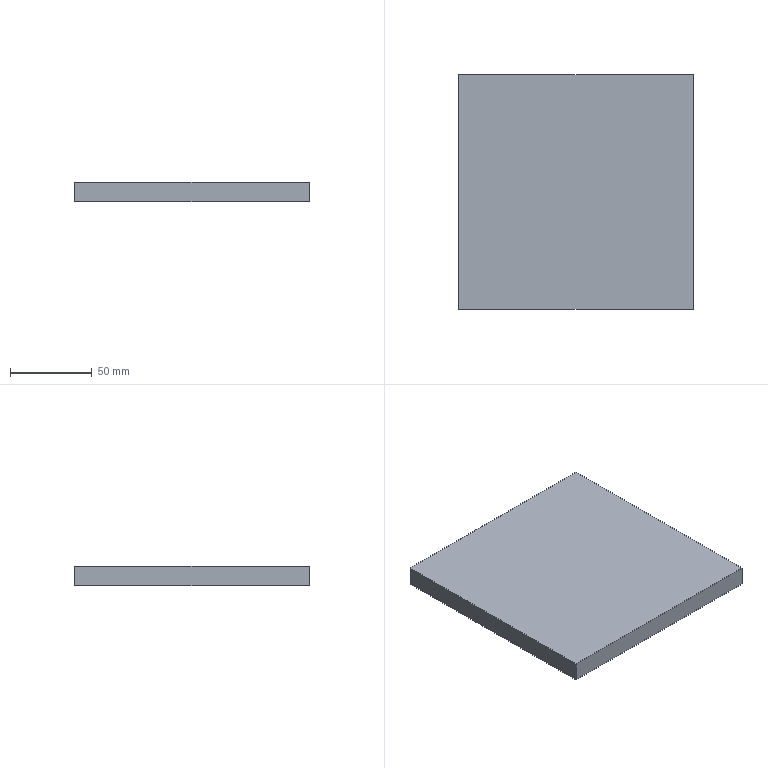Component | NX | LARGE_BASE_PLATE | 1 solid | 6 faces | box 144 x 144 x 12 mm | volume 248832 mm3 | plane 6
STEP:
#1=CARTESIAN_POINT('',(0.,0.,0.));
#2=DIRECTION('',(0.,0.,1.));
#3=DIRECTION('',(1.,0.,0.));
#4=AXIS2_PLACEMENT_3D('',#1,#2,#3);
#5=CARTESIAN_POINT('',(72.,-72.,6.));
#6=VERTEX_POINT('',#5);
#7=CARTESIAN_POINT('',(-72.,-72.,6.));
#8=VERTEX_POINT('',#7);
#9=CARTESIAN_POINT('',(0.,-72.,6.));
#10=DIRECTION('',(-1.,0.,0.));
#11=VECTOR('',#10,1.);
#12=LINE('',#9,#11);
#13=CARTESIAN_POINT('',(0.,0.,6.));
#14=DIRECTION('',(0.,0.,1.));
#15=DIRECTION('',(1.,0.,0.));
#16=AXIS2_PLACEMENT_3D('',#13,#14,#15);
#17=PLANE('',#16);
#18=CARTESIAN_POINT('',(0.,-72.));
#19=DIRECTION('',(-1.,0.));
#20=VECTOR('',#19,1.);
#21=LINE('',#18,#20);
#22=(GEOMETRIC_REPRESENTATION_CONTEXT(2)PARAMETRIC_REPRESENTATION_CONTEXT()REPRESENTATION_CONTEXT('',''));
#23=DEFINITIONAL_REPRESENTATION('',(#21),#22);
#24=PCURVE('',#17,#23);
#25=CARTESIAN_POINT('',(0.,-72.,-6.));
#26=DIRECTION('',(0.,-1.,0.));
#27=DIRECTION('',(0.,0.,-1.));
#28=AXIS2_PLACEMENT_3D('',#25,#26,#27);
#29=PLANE('',#28);
#30=CARTESIAN_POINT('',(-12.,0.));
#31=DIRECTION('',(0.,-1.));
#32=VECTOR('',#31,1.);
#33=LINE('',#30,#32);
#34=(GEOMETRIC_REPRESENTATION_CONTEXT(2)PARAMETRIC_REPRESENTATION_CONTEXT()REPRESENTATION_CONTEXT('',''));
#35=DEFINITIONAL_REPRESENTATION('',(#33),#34);
#36=PCURVE('',#29,#35);
#37=SURFACE_CURVE('',#12,(#24,#36),.PCURVE_S1.);
#38=EDGE_CURVE('',#6,#8,#37,.T.);
#39=ORIENTED_EDGE('',*,*,#38,.F.);
#40=CARTESIAN_POINT('',(72.,72.,6.));
#41=VERTEX_POINT('',#40);
#42=CARTESIAN_POINT('',(72.,0.,6.));
#43=DIRECTION('',(0.,-1.,0.));
#44=VECTOR('',#43,1.);
#45=LINE('',#42,#44);
#46=CARTESIAN_POINT('',(72.,0.));
#47=DIRECTION('',(0.,-1.));
#48=VECTOR('',#47,1.);
#49=LINE('',#46,#48);
#50=(GEOMETRIC_REPRESENTATION_CONTEXT(2)PARAMETRIC_REPRESENTATION_CONTEXT()REPRESENTATION_CONTEXT('',''));
#51=DEFINITIONAL_REPRESENTATION('',(#49),#50);
#52=PCURVE('',#17,#51);
#53=CARTESIAN_POINT('',(72.,0.,-6.));
#54=DIRECTION('',(1.,0.,0.));
#55=DIRECTION('',(0.,0.,-1.));
#56=AXIS2_PLACEMENT_3D('',#53,#54,#55);
#57=PLANE('',#56);
#58=CARTESIAN_POINT('',(-12.,0.));
#59=DIRECTION('',(0.,-1.));
#60=VECTOR('',#59,1.);
#61=LINE('',#58,#60);
#62=(GEOMETRIC_REPRESENTATION_CONTEXT(2)PARAMETRIC_REPRESENTATION_CONTEXT()REPRESENTATION_CONTEXT('',''));
#63=DEFINITIONAL_REPRESENTATION('',(#61),#62);
#64=PCURVE('',#57,#63);
#65=SURFACE_CURVE('',#45,(#52,#64),.PCURVE_S1.);
#66=EDGE_CURVE('',#41,#6,#65,.T.);
#67=ORIENTED_EDGE('',*,*,#66,.F.);
#68=CARTESIAN_POINT('',(-72.,72.,6.));
#69=VERTEX_POINT('',#68);
#70=CARTESIAN_POINT('',(0.,72.,6.));
#71=DIRECTION('',(1.,0.,0.));
#72=VECTOR('',#71,1.);
#73=LINE('',#70,#72);
#74=CARTESIAN_POINT('',(0.,72.));
#75=DIRECTION('',(1.,0.));
#76=VECTOR('',#75,1.);
#77=LINE('',#74,#76);
#78=(GEOMETRIC_REPRESENTATION_CONTEXT(2)PARAMETRIC_REPRESENTATION_CONTEXT()REPRESENTATION_CONTEXT('',''));
#79=DEFINITIONAL_REPRESENTATION('',(#77),#78);
#80=PCURVE('',#17,#79);
#81=CARTESIAN_POINT('',(0.,72.,-6.));
#82=DIRECTION('',(0.,1.,0.));
#83=DIRECTION('',(0.,0.,1.));
#84=AXIS2_PLACEMENT_3D('',#81,#82,#83);
#85=PLANE('',#84);
#86=CARTESIAN_POINT('',(12.,0.));
#87=DIRECTION('',(0.,1.));
#88=VECTOR('',#87,1.);
#89=LINE('',#86,#88);
#90=(GEOMETRIC_REPRESENTATION_CONTEXT(2)PARAMETRIC_REPRESENTATION_CONTEXT()REPRESENTATION_CONTEXT('',''));
#91=DEFINITIONAL_REPRESENTATION('',(#89),#90);
#92=PCURVE('',#85,#91);
#93=SURFACE_CURVE('',#73,(#80,#92),.PCURVE_S1.);
#94=EDGE_CURVE('',#69,#41,#93,.T.);
#95=ORIENTED_EDGE('',*,*,#94,.F.);
#96=CARTESIAN_POINT('',(-72.,0.,6.));
#97=DIRECTION('',(0.,1.,0.));
#98=VECTOR('',#97,1.);
#99=LINE('',#96,#98);
#100=CARTESIAN_POINT('',(-72.,0.));
#101=DIRECTION('',(0.,1.));
#102=VECTOR('',#101,1.);
#103=LINE('',#100,#102);
#104=(GEOMETRIC_REPRESENTATION_CONTEXT(2)PARAMETRIC_REPRESENTATION_CONTEXT()REPRESENTATION_CONTEXT('',''));
#105=DEFINITIONAL_REPRESENTATION('',(#103),#104);
#106=PCURVE('',#17,#105);
#107=CARTESIAN_POINT('',(-72.,0.,-6.));
#108=DIRECTION('',(-1.,0.,0.));
#109=DIRECTION('',(0.,0.,1.));
#110=AXIS2_PLACEMENT_3D('',#107,#108,#109);
#111=PLANE('',#110);
#112=CARTESIAN_POINT('',(12.,0.));
#113=DIRECTION('',(0.,1.));
#114=VECTOR('',#113,1.);
#115=LINE('',#112,#114);
#116=(GEOMETRIC_REPRESENTATION_CONTEXT(2)PARAMETRIC_REPRESENTATION_CONTEXT()REPRESENTATION_CONTEXT('',''));
#117=DEFINITIONAL_REPRESENTATION('',(#115),#116);
#118=PCURVE('',#111,#117);
#119=SURFACE_CURVE('',#99,(#106,#118),.PCURVE_S1.);
#120=EDGE_CURVE('',#8,#69,#119,.T.);
#121=ORIENTED_EDGE('',*,*,#120,.F.);
#122=EDGE_LOOP('',(#39,#67,#95,#121));
#123=FACE_BOUND('',#122,.T.);
#124=ADVANCED_FACE('',(#123),#17,.T.);
#125=CARTESIAN_POINT('',(72.,-72.,-6.));
#126=VERTEX_POINT('',#125);
#127=CARTESIAN_POINT('',(72.,-72.,-6.));
#128=DIRECTION('',(0.,0.,1.));
#129=VECTOR('',#128,1.);
#130=LINE('',#127,#129);
#131=CARTESIAN_POINT('',(0.,72.));
#132=DIRECTION('',(-1.,0.));
#133=VECTOR('',#132,1.);
#134=LINE('',#131,#133);
#135=(GEOMETRIC_REPRESENTATION_CONTEXT(2)PARAMETRIC_REPRESENTATION_CONTEXT()REPRESENTATION_CONTEXT('',''));
#136=DEFINITIONAL_REPRESENTATION('',(#134),#135);
#137=PCURVE('',#29,#136);
#138=CARTESIAN_POINT('',(0.,-72.));
#139=DIRECTION('',(-1.,0.));
#140=VECTOR('',#139,1.);
#141=LINE('',#138,#140);
#142=(GEOMETRIC_REPRESENTATION_CONTEXT(2)PARAMETRIC_REPRESENTATION_CONTEXT()REPRESENTATION_CONTEXT('',''));
#143=DEFINITIONAL_REPRESENTATION('',(#141),#142);
#144=PCURVE('',#57,#143);
#145=SURFACE_CURVE('',#130,(#137,#144),.PCURVE_S1.);
#146=EDGE_CURVE('',#126,#6,#145,.T.);
#147=ORIENTED_EDGE('',*,*,#146,.T.);
#148=ORIENTED_EDGE('',*,*,#38,.T.);
#149=CARTESIAN_POINT('',(-72.,-72.,-6.));
#150=VERTEX_POINT('',#149);
#151=CARTESIAN_POINT('',(-72.,-72.,-6.));
#152=DIRECTION('',(0.,0.,1.));
#153=VECTOR('',#152,1.);
#154=LINE('',#151,#153);
#155=CARTESIAN_POINT('',(0.,-72.));
#156=DIRECTION('',(-1.,0.));
#157=VECTOR('',#156,1.);
#158=LINE('',#155,#157);
#159=(GEOMETRIC_REPRESENTATION_CONTEXT(2)PARAMETRIC_REPRESENTATION_CONTEXT()REPRESENTATION_CONTEXT('',''));
#160=DEFINITIONAL_REPRESENTATION('',(#158),#159);
#161=PCURVE('',#29,#160);
#162=CARTESIAN_POINT('',(0.,-72.));
#163=DIRECTION('',(1.,0.));
#164=VECTOR('',#163,1.);
#165=LINE('',#162,#164);
#166=(GEOMETRIC_REPRESENTATION_CONTEXT(2)PARAMETRIC_REPRESENTATION_CONTEXT()REPRESENTATION_CONTEXT('',''));
#167=DEFINITIONAL_REPRESENTATION('',(#165),#166);
#168=PCURVE('',#111,#167);
#169=SURFACE_CURVE('',#154,(#161,#168),.PCURVE_S1.);
#170=EDGE_CURVE('',#150,#8,#169,.T.);
#171=ORIENTED_EDGE('',*,*,#170,.F.);
#172=CARTESIAN_POINT('',(0.,-72.,-6.));
#173=DIRECTION('',(1.,0.,0.));
#174=VECTOR('',#173,1.);
#175=LINE('',#172,#174);
#176=CARTESIAN_POINT('',(0.,0.));
#177=DIRECTION('',(0.,1.));
#178=VECTOR('',#177,1.);
#179=LINE('',#176,#178);
#180=(GEOMETRIC_REPRESENTATION_CONTEXT(2)PARAMETRIC_REPRESENTATION_CONTEXT()REPRESENTATION_CONTEXT('',''));
#181=DEFINITIONAL_REPRESENTATION('',(#179),#180);
#182=PCURVE('',#29,#181);
#183=CARTESIAN_POINT('',(0.,0.,-6.));
#184=DIRECTION('',(0.,0.,-1.));
#185=DIRECTION('',(-1.,0.,0.));
#186=AXIS2_PLACEMENT_3D('',#183,#184,#185);
#187=PLANE('',#186);
#188=CARTESIAN_POINT('',(0.,-72.));
#189=DIRECTION('',(-1.,0.));
#190=VECTOR('',#189,1.);
#191=LINE('',#188,#190);
#192=(GEOMETRIC_REPRESENTATION_CONTEXT(2)PARAMETRIC_REPRESENTATION_CONTEXT()REPRESENTATION_CONTEXT('',''));
#193=DEFINITIONAL_REPRESENTATION('',(#191),#192);
#194=PCURVE('',#187,#193);
#195=SURFACE_CURVE('',#175,(#182,#194),.PCURVE_S1.);
#196=EDGE_CURVE('',#150,#126,#195,.T.);
#197=ORIENTED_EDGE('',*,*,#196,.T.);
#198=EDGE_LOOP('',(#147,#148,#171,#197));
#199=FACE_BOUND('',#198,.T.);
#200=ADVANCED_FACE('',(#199),#29,.T.);
#201=ORIENTED_EDGE('',*,*,#170,.T.);
#202=ORIENTED_EDGE('',*,*,#120,.T.);
#203=CARTESIAN_POINT('',(-72.,72.,-6.));
#204=VERTEX_POINT('',#203);
#205=CARTESIAN_POINT('',(-72.,72.,-6.));
#206=DIRECTION('',(0.,0.,1.));
#207=VECTOR('',#206,1.);
#208=LINE('',#205,#207);
#209=CARTESIAN_POINT('',(0.,72.));
#210=DIRECTION('',(1.,0.));
#211=VECTOR('',#210,1.);
#212=LINE('',#209,#211);
#213=(GEOMETRIC_REPRESENTATION_CONTEXT(2)PARAMETRIC_REPRESENTATION_CONTEXT()REPRESENTATION_CONTEXT('',''));
#214=DEFINITIONAL_REPRESENTATION('',(#212),#213);
#215=PCURVE('',#111,#214);
#216=CARTESIAN_POINT('',(0.,-72.));
#217=DIRECTION('',(1.,0.));
#218=VECTOR('',#217,1.);
#219=LINE('',#216,#218);
#220=(GEOMETRIC_REPRESENTATION_CONTEXT(2)PARAMETRIC_REPRESENTATION_CONTEXT()REPRESENTATION_CONTEXT('',''));
#221=DEFINITIONAL_REPRESENTATION('',(#219),#220);
#222=PCURVE('',#85,#221);
#223=SURFACE_CURVE('',#208,(#215,#222),.PCURVE_S1.);
#224=EDGE_CURVE('',#204,#69,#223,.T.);
#225=ORIENTED_EDGE('',*,*,#224,.F.);
#226=CARTESIAN_POINT('',(-72.,0.,-6.));
#227=DIRECTION('',(0.,-1.,0.));
#228=VECTOR('',#227,1.);
#229=LINE('',#226,#228);
#230=CARTESIAN_POINT('',(0.,0.));
#231=DIRECTION('',(0.,-1.));
#232=VECTOR('',#231,1.);
#233=LINE('',#230,#232);
#234=(GEOMETRIC_REPRESENTATION_CONTEXT(2)PARAMETRIC_REPRESENTATION_CONTEXT()REPRESENTATION_CONTEXT('',''));
#235=DEFINITIONAL_REPRESENTATION('',(#233),#234);
#236=PCURVE('',#111,#235);
#237=CARTESIAN_POINT('',(72.,0.));
#238=DIRECTION('',(0.,-1.));
#239=VECTOR('',#238,1.);
#240=LINE('',#237,#239);
#241=(GEOMETRIC_REPRESENTATION_CONTEXT(2)PARAMETRIC_REPRESENTATION_CONTEXT()REPRESENTATION_CONTEXT('',''));
#242=DEFINITIONAL_REPRESENTATION('',(#240),#241);
#243=PCURVE('',#187,#242);
#244=SURFACE_CURVE('',#229,(#236,#243),.PCURVE_S1.);
#245=EDGE_CURVE('',#204,#150,#244,.T.);
#246=ORIENTED_EDGE('',*,*,#245,.T.);
#247=EDGE_LOOP('',(#201,#202,#225,#246));
#248=FACE_BOUND('',#247,.T.);
#249=ADVANCED_FACE('',(#248),#111,.T.);
#250=ORIENTED_EDGE('',*,*,#224,.T.);
#251=ORIENTED_EDGE('',*,*,#94,.T.);
#252=CARTESIAN_POINT('',(72.,72.,-6.));
#253=VERTEX_POINT('',#252);
#254=CARTESIAN_POINT('',(72.,72.,-6.));
#255=DIRECTION('',(0.,0.,1.));
#256=VECTOR('',#255,1.);
#257=LINE('',#254,#256);
#258=CARTESIAN_POINT('',(0.,72.));
#259=DIRECTION('',(1.,0.));
#260=VECTOR('',#259,1.);
#261=LINE('',#258,#260);
#262=(GEOMETRIC_REPRESENTATION_CONTEXT(2)PARAMETRIC_REPRESENTATION_CONTEXT()REPRESENTATION_CONTEXT('',''));
#263=DEFINITIONAL_REPRESENTATION('',(#261),#262);
#264=PCURVE('',#85,#263);
#265=CARTESIAN_POINT('',(0.,72.));
#266=DIRECTION('',(-1.,0.));
#267=VECTOR('',#266,1.);
#268=LINE('',#265,#267);
#269=(GEOMETRIC_REPRESENTATION_CONTEXT(2)PARAMETRIC_REPRESENTATION_CONTEXT()REPRESENTATION_CONTEXT('',''));
#270=DEFINITIONAL_REPRESENTATION('',(#268),#269);
#271=PCURVE('',#57,#270);
#272=SURFACE_CURVE('',#257,(#264,#271),.PCURVE_S1.);
#273=EDGE_CURVE('',#253,#41,#272,.T.);
#274=ORIENTED_EDGE('',*,*,#273,.F.);
#275=CARTESIAN_POINT('',(0.,72.,-6.));
#276=DIRECTION('',(-1.,0.,0.));
#277=VECTOR('',#276,1.);
#278=LINE('',#275,#277);
#279=CARTESIAN_POINT('',(0.,0.));
#280=DIRECTION('',(0.,-1.));
#281=VECTOR('',#280,1.);
#282=LINE('',#279,#281);
#283=(GEOMETRIC_REPRESENTATION_CONTEXT(2)PARAMETRIC_REPRESENTATION_CONTEXT()REPRESENTATION_CONTEXT('',''));
#284=DEFINITIONAL_REPRESENTATION('',(#282),#283);
#285=PCURVE('',#85,#284);
#286=CARTESIAN_POINT('',(0.,72.));
#287=DIRECTION('',(1.,0.));
#288=VECTOR('',#287,1.);
#289=LINE('',#286,#288);
#290=(GEOMETRIC_REPRESENTATION_CONTEXT(2)PARAMETRIC_REPRESENTATION_CONTEXT()REPRESENTATION_CONTEXT('',''));
#291=DEFINITIONAL_REPRESENTATION('',(#289),#290);
#292=PCURVE('',#187,#291);
#293=SURFACE_CURVE('',#278,(#285,#292),.PCURVE_S1.);
#294=EDGE_CURVE('',#253,#204,#293,.T.);
#295=ORIENTED_EDGE('',*,*,#294,.T.);
#296=EDGE_LOOP('',(#250,#251,#274,#295));
#297=FACE_BOUND('',#296,.T.);
#298=ADVANCED_FACE('',(#297),#85,.T.);
#299=CARTESIAN_POINT('',(72.,0.,-6.));
#300=DIRECTION('',(0.,1.,0.));
#301=VECTOR('',#300,1.);
#302=LINE('',#299,#301);
#303=CARTESIAN_POINT('',(-72.,0.));
#304=DIRECTION('',(0.,1.));
#305=VECTOR('',#304,1.);
#306=LINE('',#303,#305);
#307=(GEOMETRIC_REPRESENTATION_CONTEXT(2)PARAMETRIC_REPRESENTATION_CONTEXT()REPRESENTATION_CONTEXT('',''));
#308=DEFINITIONAL_REPRESENTATION('',(#306),#307);
#309=PCURVE('',#187,#308);
#310=CARTESIAN_POINT('',(0.,0.));
#311=DIRECTION('',(0.,1.));
#312=VECTOR('',#311,1.);
#313=LINE('',#310,#312);
#314=(GEOMETRIC_REPRESENTATION_CONTEXT(2)PARAMETRIC_REPRESENTATION_CONTEXT()REPRESENTATION_CONTEXT('',''));
#315=DEFINITIONAL_REPRESENTATION('',(#313),#314);
#316=PCURVE('',#57,#315);
#317=SURFACE_CURVE('',#302,(#309,#316),.PCURVE_S1.);
#318=EDGE_CURVE('',#126,#253,#317,.T.);
#319=ORIENTED_EDGE('',*,*,#318,.F.);
#320=ORIENTED_EDGE('',*,*,#196,.F.);
#321=ORIENTED_EDGE('',*,*,#245,.F.);
#322=ORIENTED_EDGE('',*,*,#294,.F.);
#323=EDGE_LOOP('',(#319,#320,#321,#322));
#324=FACE_BOUND('',#323,.T.);
#325=ADVANCED_FACE('',(#324),#187,.T.);
#326=ORIENTED_EDGE('',*,*,#318,.T.);
#327=ORIENTED_EDGE('',*,*,#273,.T.);
#328=ORIENTED_EDGE('',*,*,#66,.T.);
#329=ORIENTED_EDGE('',*,*,#146,.F.);
#330=EDGE_LOOP('',(#326,#327,#328,#329));
#331=FACE_BOUND('',#330,.T.);
#332=ADVANCED_FACE('',(#331),#57,.T.);
#333=CLOSED_SHELL('',(#124,#200,#249,#298,#325,#332));
#334=MANIFOLD_SOLID_BREP('',#333);
#335=(LENGTH_UNIT()NAMED_UNIT(*)SI_UNIT(.MILLI.,.METRE.));
#336=UNCERTAINTY_MEASURE_WITH_UNIT(LENGTH_MEASURE(0.0000001),#335,'','');
#337=(NAMED_UNIT(*)PLANE_ANGLE_UNIT()SI_UNIT($,.RADIAN.));
#338=(NAMED_UNIT(*)SI_UNIT($,.STERADIAN.)SOLID_ANGLE_UNIT());
#339=(GEOMETRIC_REPRESENTATION_CONTEXT(3)GLOBAL_UNCERTAINTY_ASSIGNED_CONTEXT((#336))GLOBAL_UNIT_ASSIGNED_CONTEXT((#335,#337,#338))REPRESENTATION_CONTEXT('',''));
#340=ADVANCED_BREP_SHAPE_REPRESENTATION('',(#4,#334),#339);